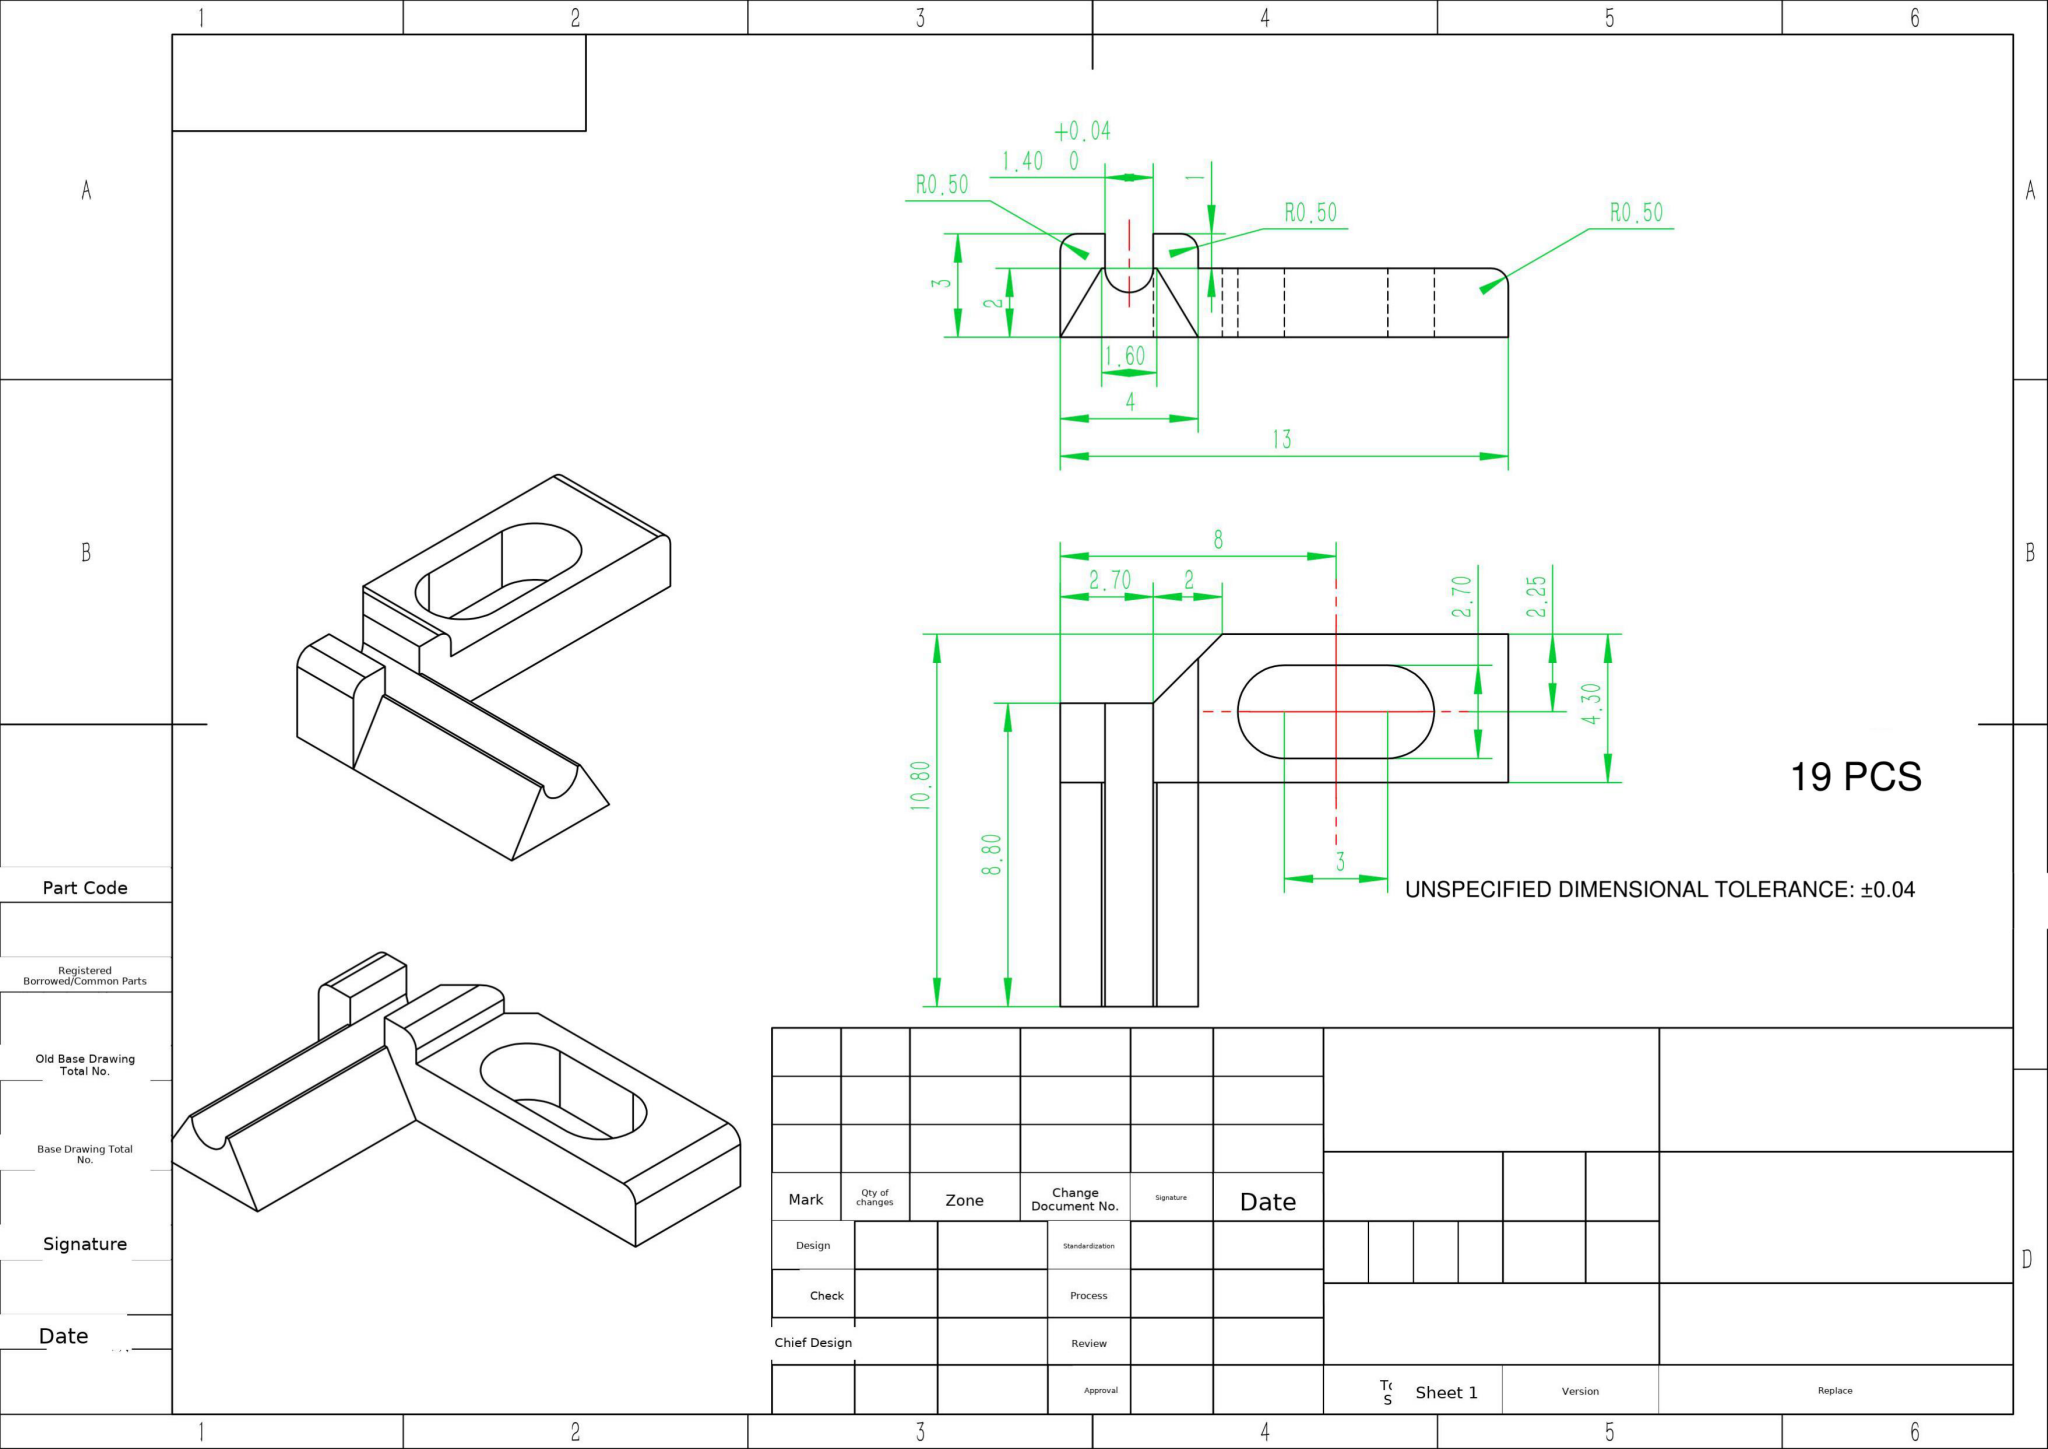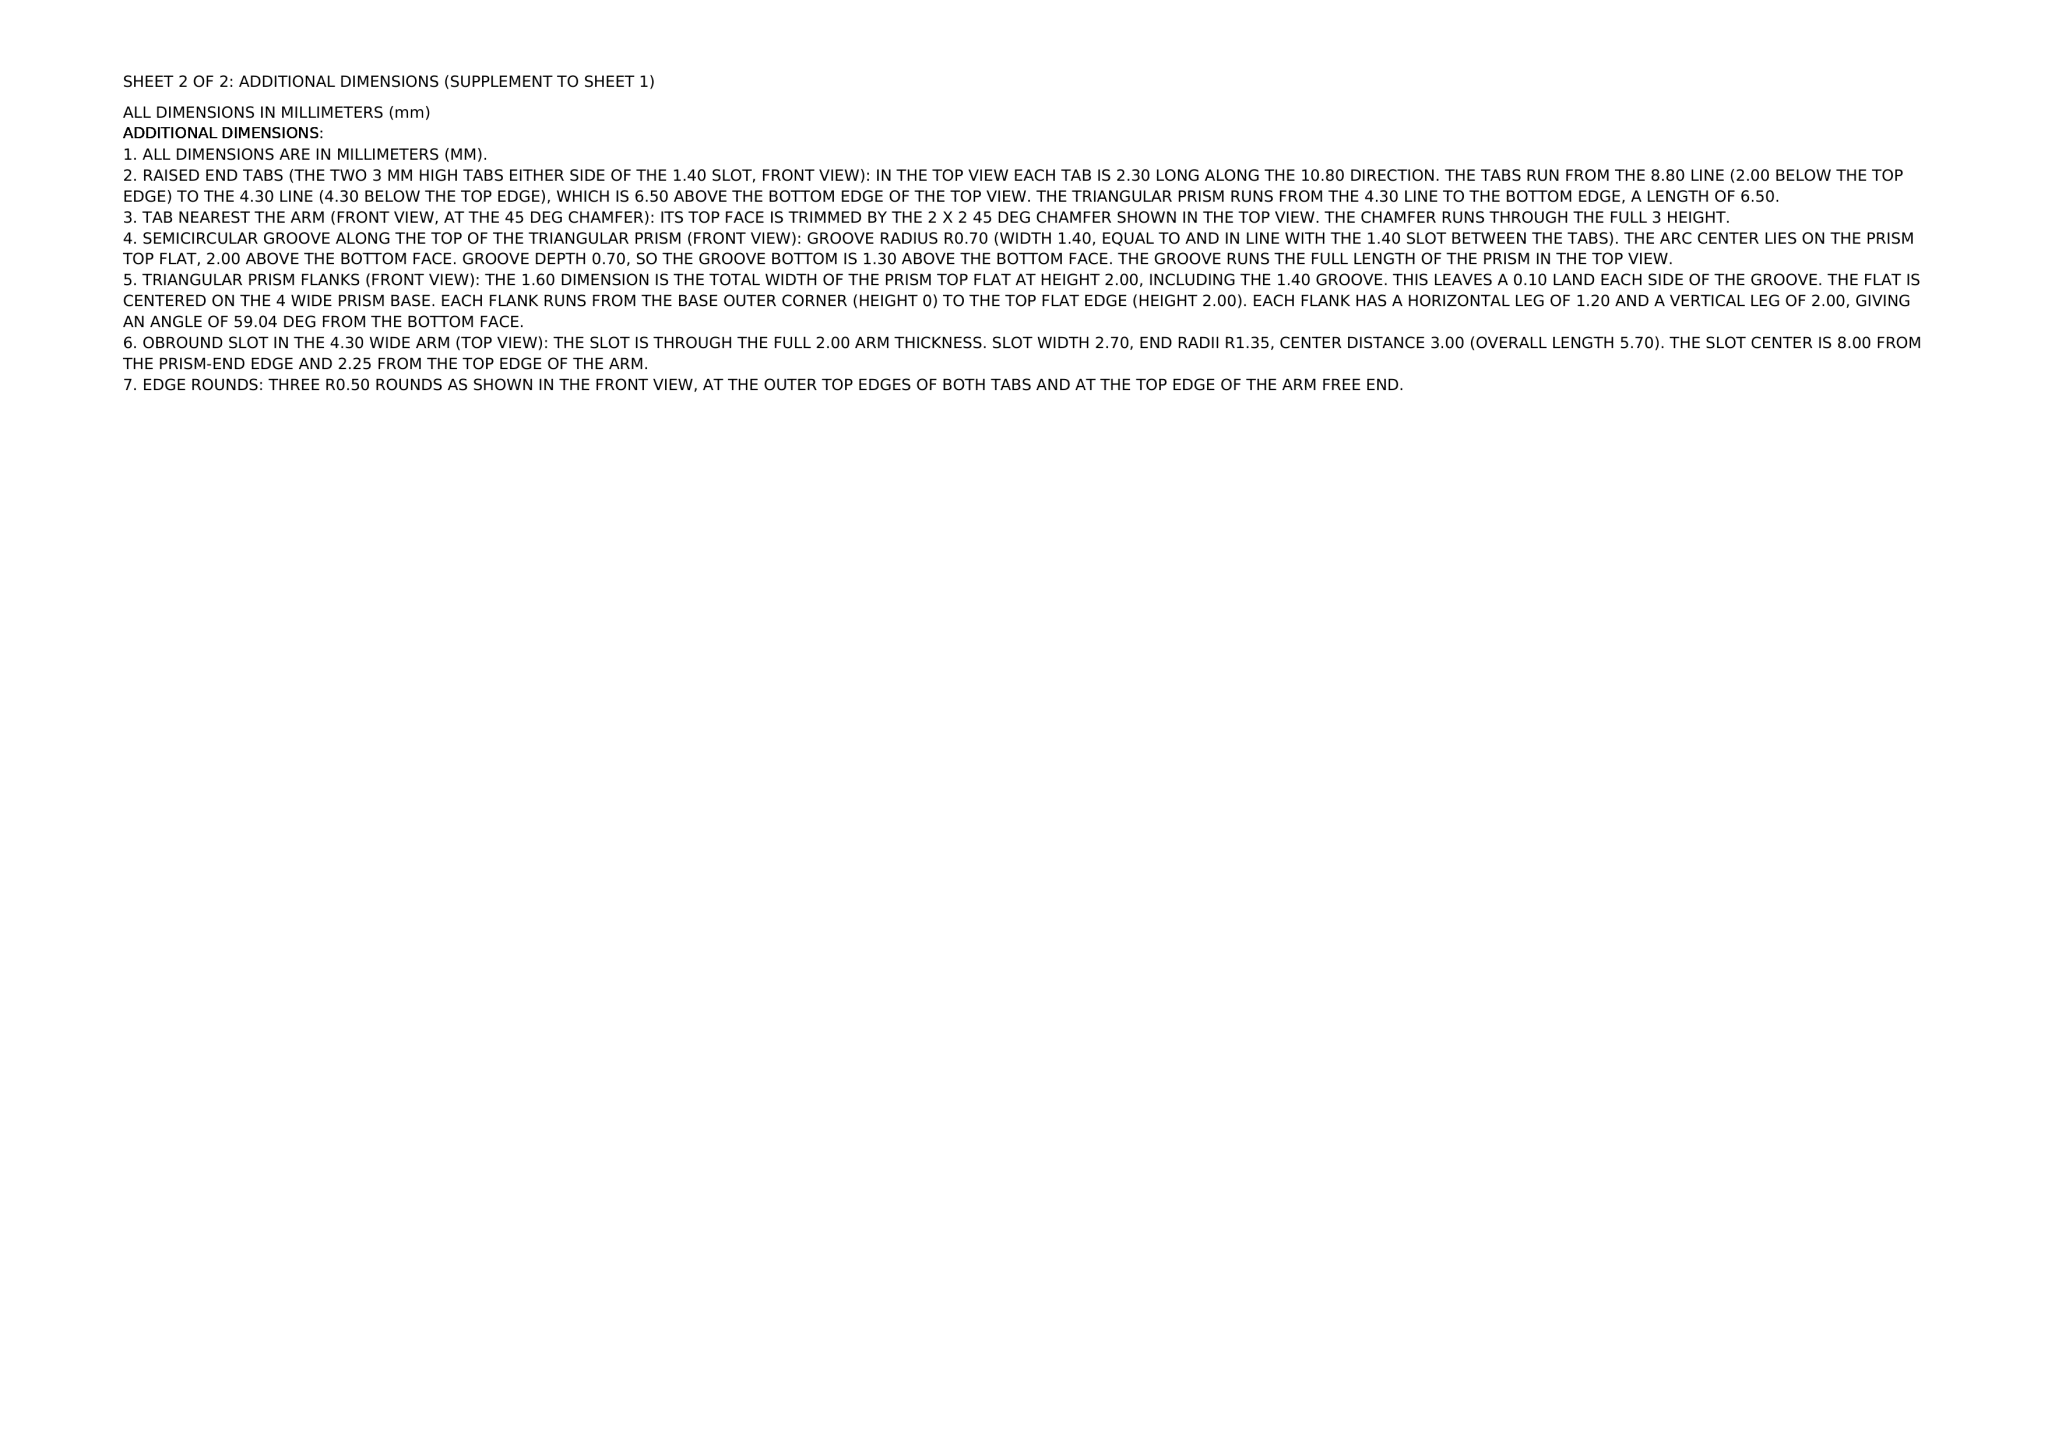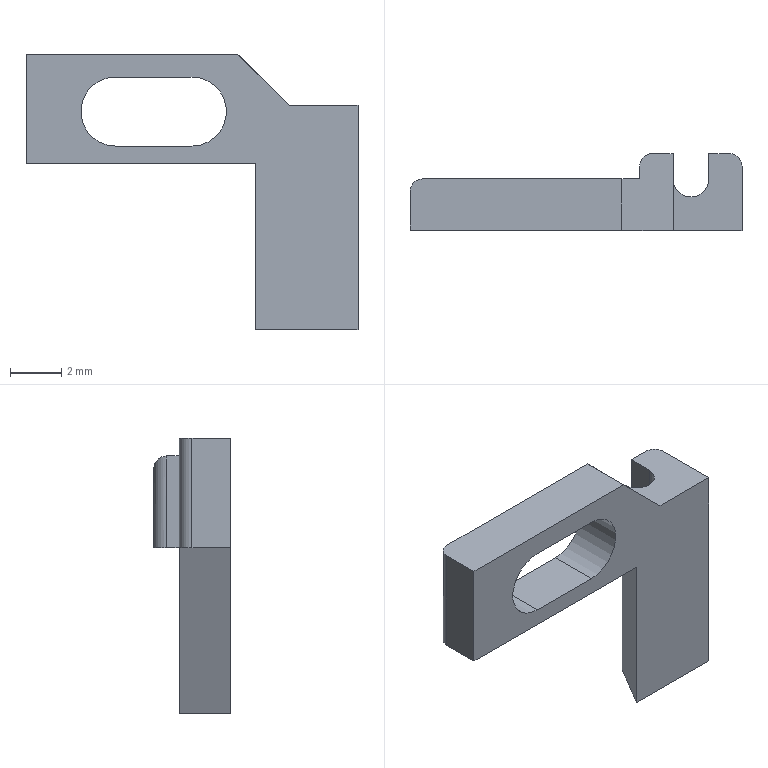Part | NX | mm | Offset Pedestal Clevis Bracket | 1 solid | 27 faces | box 13 x 3 x 10.8 mm | volume 105 mm3 | plane 21 | cylinder 6 | commonest cylinder face diameters 1 x3 2.7 x2 1.4 x1
STEP:
#1=COLOUR_RGB('',0.8431,0.,0.08627);
#2=FILL_AREA_STYLE_COLOUR('',#1);
#3=FILL_AREA_STYLE('',(#2));
#4=SURFACE_STYLE_FILL_AREA(#3);
#5=SURFACE_SIDE_STYLE('',(#4));
#6=SURFACE_STYLE_USAGE(.BOTH.,#5);
#7=PRESENTATION_STYLE_ASSIGNMENT((#6));
#8=CARTESIAN_POINT('',(9.,2.,-4.3));
#9=VERTEX_POINT('',#8);
#10=CARTESIAN_POINT('',(9.,2.5,-4.3));
#11=VERTEX_POINT('',#10);
#12=CARTESIAN_POINT('',(9.,2.,-4.3));
#13=DIRECTION('',(0.,1.,0.));
#14=VECTOR('',#13,1000.);
#15=LINE('',#12,#14);
#16=EDGE_CURVE('',#9,#11,#15,.T.);
#17=ORIENTED_EDGE('',*,*,#16,.T.);
#18=CARTESIAN_POINT('',(9.5,3.,-4.3));
#19=VERTEX_POINT('',#18);
#20=CARTESIAN_POINT('',(9.5,2.5,-4.3));
#21=DIRECTION('',(0.,0.,-1.));
#22=DIRECTION('',(1.,0.,0.));
#23=AXIS2_PLACEMENT_3D('',#20,#21,#22);
#24=CIRCLE('',#23,0.5);
#25=EDGE_CURVE('',#11,#19,#24,.T.);
#26=ORIENTED_EDGE('',*,*,#25,.T.);
#27=CARTESIAN_POINT('',(10.3,3.,-4.3));
#28=VERTEX_POINT('',#27);
#29=CARTESIAN_POINT('',(0.,3.,-4.3));
#30=DIRECTION('',(-1.,0.,0.));
#31=VECTOR('',#30,1000.);
#32=LINE('',#29,#31);
#33=EDGE_CURVE('',#28,#19,#32,.T.);
#34=ORIENTED_EDGE('',*,*,#33,.F.);
#35=CARTESIAN_POINT('',(10.3,2.,-4.3));
#36=VERTEX_POINT('',#35);
#37=CARTESIAN_POINT('',(10.3,2.,-4.3));
#38=DIRECTION('',(0.,-1.,0.));
#39=VECTOR('',#38,1000.);
#40=LINE('',#37,#39);
#41=EDGE_CURVE('',#28,#36,#40,.T.);
#42=ORIENTED_EDGE('',*,*,#41,.T.);
#43=CARTESIAN_POINT('',(10.2,2.,-4.3));
#44=VERTEX_POINT('',#43);
#45=CARTESIAN_POINT('',(0.,2.,-4.3));
#46=DIRECTION('',(-1.,0.,0.));
#47=VECTOR('',#46,1000.);
#48=LINE('',#45,#47);
#49=EDGE_CURVE('',#36,#44,#48,.T.);
#50=ORIENTED_EDGE('',*,*,#49,.T.);
#51=CARTESIAN_POINT('',(9.,0.,-4.3));
#52=VERTEX_POINT('',#51);
#53=CARTESIAN_POINT('',(7.5,-2.5,-4.3));
#54=DIRECTION('',(-0.5145,-0.8575,0.));
#55=VECTOR('',#54,1000.);
#56=LINE('',#53,#55);
#57=EDGE_CURVE('',#44,#52,#56,.T.);
#58=ORIENTED_EDGE('',*,*,#57,.T.);
#59=CARTESIAN_POINT('',(0.,0.,-4.3));
#60=VERTEX_POINT('',#59);
#61=CARTESIAN_POINT('',(0.,0.,-4.3));
#62=DIRECTION('',(-1.,0.,0.));
#63=VECTOR('',#62,1000.);
#64=LINE('',#61,#63);
#65=EDGE_CURVE('',#52,#60,#64,.T.);
#66=ORIENTED_EDGE('',*,*,#65,.T.);
#67=CARTESIAN_POINT('',(0.,1.5,-4.3));
#68=VERTEX_POINT('',#67);
#69=CARTESIAN_POINT('',(0.,2.,-4.3));
#70=DIRECTION('',(0.,-1.,0.));
#71=VECTOR('',#70,1000.);
#72=LINE('',#69,#71);
#73=EDGE_CURVE('',#68,#60,#72,.T.);
#74=ORIENTED_EDGE('',*,*,#73,.F.);
#75=CARTESIAN_POINT('',(0.5,2.,-4.3));
#76=VERTEX_POINT('',#75);
#77=CARTESIAN_POINT('',(0.5,1.5,-4.3));
#78=DIRECTION('',(0.,0.,-1.));
#79=DIRECTION('',(1.,0.,0.));
#80=AXIS2_PLACEMENT_3D('',#77,#78,#79);
#81=CIRCLE('',#80,0.5);
#82=EDGE_CURVE('',#68,#76,#81,.T.);
#83=ORIENTED_EDGE('',*,*,#82,.T.);
#84=CARTESIAN_POINT('',(0.,2.,-4.3));
#85=DIRECTION('',(-1.,0.,0.));
#86=VECTOR('',#85,1000.);
#87=LINE('',#84,#86);
#88=EDGE_CURVE('',#9,#76,#87,.T.);
#89=ORIENTED_EDGE('',*,*,#88,.F.);
#90=EDGE_LOOP('',(#17,#26,#34,#42,#50,#58,#66,#74,#83,#89));
#91=FACE_OUTER_BOUND('',#90,.T.);
#92=CARTESIAN_POINT('',(0.,2.,-4.3));
#93=DIRECTION('',(0.,0.,1.));
#94=DIRECTION('',(1.,0.,0.));
#95=AXIS2_PLACEMENT_3D('',#92,#93,#94);
#96=PLANE('',#95);
#97=ADVANCED_FACE('',(#91),#96,.F.);
#98=ORIENTED_EDGE('',*,*,#33,.T.);
#99=CARTESIAN_POINT('',(9.5,3.,-1.2));
#100=VERTEX_POINT('',#99);
#101=CARTESIAN_POINT('',(9.5,3.,-0.7));
#102=DIRECTION('',(0.,0.,1.));
#103=VECTOR('',#102,1000.);
#104=LINE('',#101,#103);
#105=EDGE_CURVE('',#19,#100,#104,.T.);
#106=ORIENTED_EDGE('',*,*,#105,.T.);
#107=CARTESIAN_POINT('',(10.3,3.,-2.));
#108=VERTEX_POINT('',#107);
#109=CARTESIAN_POINT('',(8.3,3.,0.));
#110=DIRECTION('',(0.7071,0.,-0.7071));
#111=VECTOR('',#110,1000.);
#112=LINE('',#109,#111);
#113=EDGE_CURVE('',#100,#108,#112,.T.);
#114=ORIENTED_EDGE('',*,*,#113,.T.);
#115=CARTESIAN_POINT('',(10.3,3.,-8.));
#116=DIRECTION('',(0.,0.,1.));
#117=VECTOR('',#116,1000.);
#118=LINE('',#115,#117);
#119=EDGE_CURVE('',#28,#108,#118,.T.);
#120=ORIENTED_EDGE('',*,*,#119,.F.);
#121=EDGE_LOOP('',(#98,#106,#114,#120));
#122=FACE_OUTER_BOUND('',#121,.T.);
#123=CARTESIAN_POINT('',(0.,3.,0.));
#124=DIRECTION('',(0.,1.,0.));
#125=DIRECTION('',(0.,0.,1.));
#126=AXIS2_PLACEMENT_3D('',#123,#124,#125);
#127=PLANE('',#126);
#128=ADVANCED_FACE('',(#122),#127,.T.);
#129=CARTESIAN_POINT('',(11.8,2.,-4.3));
#130=VERTEX_POINT('',#129);
#131=CARTESIAN_POINT('',(11.7,2.,-4.3));
#132=VERTEX_POINT('',#131);
#133=CARTESIAN_POINT('',(0.,2.,-4.3));
#134=DIRECTION('',(-1.,0.,0.));
#135=VECTOR('',#134,1000.);
#136=LINE('',#133,#135);
#137=EDGE_CURVE('',#130,#132,#136,.T.);
#138=ORIENTED_EDGE('',*,*,#137,.F.);
#139=CARTESIAN_POINT('',(11.8,2.,-10.8));
#140=VERTEX_POINT('',#139);
#141=CARTESIAN_POINT('',(11.8,2.,-0.));
#142=DIRECTION('',(-0.,0.,-1.));
#143=VECTOR('',#142,1000.);
#144=LINE('',#141,#143);
#145=EDGE_CURVE('',#130,#140,#144,.T.);
#146=ORIENTED_EDGE('',*,*,#145,.T.);
#147=CARTESIAN_POINT('',(11.7,2.,-10.8));
#148=VERTEX_POINT('',#147);
#149=CARTESIAN_POINT('',(11.7,2.,-10.8));
#150=DIRECTION('',(1.,0.,0.));
#151=VECTOR('',#150,1000.);
#152=LINE('',#149,#151);
#153=EDGE_CURVE('',#148,#140,#152,.T.);
#154=ORIENTED_EDGE('',*,*,#153,.F.);
#155=CARTESIAN_POINT('',(11.7,2.,5.7));
#156=DIRECTION('',(0.,0.,-1.));
#157=VECTOR('',#156,1000.);
#158=LINE('',#155,#157);
#159=EDGE_CURVE('',#132,#148,#158,.T.);
#160=ORIENTED_EDGE('',*,*,#159,.F.);
#161=EDGE_LOOP('',(#138,#146,#154,#160));
#162=FACE_OUTER_BOUND('',#161,.T.);
#163=CARTESIAN_POINT('',(0.,2.,0.));
#164=DIRECTION('',(0.,-1.,0.));
#165=DIRECTION('',(0.,0.,-1.));
#166=AXIS2_PLACEMENT_3D('',#163,#164,#165);
#167=PLANE('',#166);
#168=ADVANCED_FACE('',(#162),#167,.F.);
#169=CARTESIAN_POINT('',(10.2,2.,-10.8));
#170=VERTEX_POINT('',#169);
#171=CARTESIAN_POINT('',(10.3,2.,-10.8));
#172=VERTEX_POINT('',#171);
#173=CARTESIAN_POINT('',(9.,2.,-10.8));
#174=DIRECTION('',(1.,-0.,0.));
#175=VECTOR('',#174,1000.);
#176=LINE('',#173,#175);
#177=EDGE_CURVE('',#170,#172,#176,.T.);
#178=ORIENTED_EDGE('',*,*,#177,.F.);
#179=CARTESIAN_POINT('',(10.2,2.,0.));
#180=DIRECTION('',(0.,0.,1.));
#181=VECTOR('',#180,1000.);
#182=LINE('',#179,#181);
#183=EDGE_CURVE('',#170,#44,#182,.T.);
#184=ORIENTED_EDGE('',*,*,#183,.T.);
#185=ORIENTED_EDGE('',*,*,#49,.F.);
#186=CARTESIAN_POINT('',(10.3,2.,5.7));
#187=DIRECTION('',(0.,0.,-1.));
#188=VECTOR('',#187,1000.);
#189=LINE('',#186,#188);
#190=EDGE_CURVE('',#36,#172,#189,.T.);
#191=ORIENTED_EDGE('',*,*,#190,.T.);
#192=EDGE_LOOP('',(#178,#184,#185,#191));
#193=FACE_OUTER_BOUND('',#192,.T.);
#194=CARTESIAN_POINT('',(0.,2.,0.));
#195=DIRECTION('',(0.,-1.,0.));
#196=DIRECTION('',(0.,0.,-1.));
#197=AXIS2_PLACEMENT_3D('',#194,#195,#196);
#198=PLANE('',#197);
#199=ADVANCED_FACE('',(#193),#198,.F.);
#200=CARTESIAN_POINT('',(12.5,3.,-4.3));
#201=VERTEX_POINT('',#200);
#202=CARTESIAN_POINT('',(11.7,3.,-4.3));
#203=VERTEX_POINT('',#202);
#204=CARTESIAN_POINT('',(0.,3.,-4.3));
#205=DIRECTION('',(-1.,0.,0.));
#206=VECTOR('',#205,1000.);
#207=LINE('',#204,#206);
#208=EDGE_CURVE('',#201,#203,#207,.T.);
#209=ORIENTED_EDGE('',*,*,#208,.F.);
#210=CARTESIAN_POINT('',(13.,2.5,-4.3));
#211=VERTEX_POINT('',#210);
#212=CARTESIAN_POINT('',(12.5,2.5,-4.3));
#213=DIRECTION('',(0.,0.,-1.));
#214=DIRECTION('',(1.,0.,0.));
#215=AXIS2_PLACEMENT_3D('',#212,#213,#214);
#216=CIRCLE('',#215,0.5);
#217=EDGE_CURVE('',#201,#211,#216,.T.);
#218=ORIENTED_EDGE('',*,*,#217,.T.);
#219=CARTESIAN_POINT('',(13.,0.,-4.3));
#220=VERTEX_POINT('',#219);
#221=CARTESIAN_POINT('',(13.,3.,-4.3));
#222=DIRECTION('',(0.,-1.,0.));
#223=VECTOR('',#222,1000.);
#224=LINE('',#221,#223);
#225=EDGE_CURVE('',#211,#220,#224,.T.);
#226=ORIENTED_EDGE('',*,*,#225,.T.);
#227=CARTESIAN_POINT('',(8.676,7.206,-4.3));
#228=DIRECTION('',(-0.5145,0.8575,0.));
#229=VECTOR('',#228,1000.);
#230=LINE('',#227,#229);
#231=EDGE_CURVE('',#220,#130,#230,.T.);
#232=ORIENTED_EDGE('',*,*,#231,.T.);
#233=ORIENTED_EDGE('',*,*,#137,.T.);
#234=CARTESIAN_POINT('',(11.7,2.,-4.3));
#235=DIRECTION('',(0.,1.,0.));
#236=VECTOR('',#235,1000.);
#237=LINE('',#234,#236);
#238=EDGE_CURVE('',#132,#203,#237,.T.);
#239=ORIENTED_EDGE('',*,*,#238,.T.);
#240=EDGE_LOOP('',(#209,#218,#226,#232,#233,#239));
#241=FACE_OUTER_BOUND('',#240,.T.);
#242=CARTESIAN_POINT('',(0.,2.,-4.3));
#243=DIRECTION('',(0.,0.,1.));
#244=DIRECTION('',(1.,0.,0.));
#245=AXIS2_PLACEMENT_3D('',#242,#243,#244);
#246=PLANE('',#245);
#247=ADVANCED_FACE('',(#241),#246,.F.);
#248=CARTESIAN_POINT('',(0.,1.5,0.));
#249=VERTEX_POINT('',#248);
#250=CARTESIAN_POINT('',(0.,0.,0.));
#251=VERTEX_POINT('',#250);
#252=CARTESIAN_POINT('',(0.,2.,0.));
#253=DIRECTION('',(0.,-1.,0.));
#254=VECTOR('',#253,1000.);
#255=LINE('',#252,#254);
#256=EDGE_CURVE('',#249,#251,#255,.T.);
#257=ORIENTED_EDGE('',*,*,#256,.F.);
#258=CARTESIAN_POINT('',(0.,1.5,0.));
#259=DIRECTION('',(0.,0.,-1.));
#260=VECTOR('',#259,1000.);
#261=LINE('',#258,#260);
#262=EDGE_CURVE('',#249,#68,#261,.T.);
#263=ORIENTED_EDGE('',*,*,#262,.T.);
#264=ORIENTED_EDGE('',*,*,#73,.T.);
#265=CARTESIAN_POINT('',(0.,0.,0.));
#266=DIRECTION('',(0.,0.,1.));
#267=VECTOR('',#266,1000.);
#268=LINE('',#265,#267);
#269=EDGE_CURVE('',#60,#251,#268,.T.);
#270=ORIENTED_EDGE('',*,*,#269,.T.);
#271=EDGE_LOOP('',(#257,#263,#264,#270));
#272=FACE_OUTER_BOUND('',#271,.T.);
#273=CARTESIAN_POINT('',(0.,2.,0.));
#274=DIRECTION('',(1.,0.,0.));
#275=DIRECTION('',(0.,0.,-1.));
#276=AXIS2_PLACEMENT_3D('',#273,#274,#275);
#277=PLANE('',#276);
#278=ADVANCED_FACE('',(#272),#277,.F.);
#279=CARTESIAN_POINT('',(0.5,2.,0.));
#280=VERTEX_POINT('',#279);
#281=CARTESIAN_POINT('',(8.3,2.,0.));
#282=VERTEX_POINT('',#281);
#283=CARTESIAN_POINT('',(0.,2.,0.));
#284=DIRECTION('',(1.,0.,0.));
#285=VECTOR('',#284,1000.);
#286=LINE('',#283,#285);
#287=EDGE_CURVE('',#280,#282,#286,.T.);
#288=ORIENTED_EDGE('',*,*,#287,.F.);
#289=CARTESIAN_POINT('',(0.5,1.5,0.));
#290=DIRECTION('',(0.,0.,1.));
#291=DIRECTION('',(-1.,0.,0.));
#292=AXIS2_PLACEMENT_3D('',#289,#290,#291);
#293=CIRCLE('',#292,0.5);
#294=EDGE_CURVE('',#280,#249,#293,.T.);
#295=ORIENTED_EDGE('',*,*,#294,.T.);
#296=ORIENTED_EDGE('',*,*,#256,.T.);
#297=CARTESIAN_POINT('',(8.3,0.,0.));
#298=VERTEX_POINT('',#297);
#299=CARTESIAN_POINT('',(0.,0.,0.));
#300=DIRECTION('',(1.,0.,0.));
#301=VECTOR('',#300,1000.);
#302=LINE('',#299,#301);
#303=EDGE_CURVE('',#251,#298,#302,.T.);
#304=ORIENTED_EDGE('',*,*,#303,.T.);
#305=CARTESIAN_POINT('',(8.3,2.,0.));
#306=DIRECTION('',(0.,1.,0.));
#307=VECTOR('',#306,1000.);
#308=LINE('',#305,#307);
#309=EDGE_CURVE('',#298,#282,#308,.T.);
#310=ORIENTED_EDGE('',*,*,#309,.T.);
#311=EDGE_LOOP('',(#288,#295,#296,#304,#310));
#312=FACE_OUTER_BOUND('',#311,.T.);
#313=CARTESIAN_POINT('',(0.,2.,0.));
#314=DIRECTION('',(0.,0.,-1.));
#315=DIRECTION('',(-1.,0.,0.));
#316=AXIS2_PLACEMENT_3D('',#313,#314,#315);
#317=PLANE('',#316);
#318=ADVANCED_FACE('',(#312),#317,.F.);
#319=CARTESIAN_POINT('',(13.,0.,-2.));
#320=VERTEX_POINT('',#319);
#321=CARTESIAN_POINT('',(13.,0.,-0.));
#322=DIRECTION('',(-0.,0.,-1.));
#323=VECTOR('',#322,1000.);
#324=LINE('',#321,#323);
#325=EDGE_CURVE('',#320,#220,#324,.T.);
#326=ORIENTED_EDGE('',*,*,#325,.F.);
#327=CARTESIAN_POINT('',(10.3,0.,-2.));
#328=VERTEX_POINT('',#327);
#329=CARTESIAN_POINT('',(-0.,0.,-2.));
#330=DIRECTION('',(1.,0.,-0.));
#331=VECTOR('',#330,1000.);
#332=LINE('',#329,#331);
#333=EDGE_CURVE('',#328,#320,#332,.T.);
#334=ORIENTED_EDGE('',*,*,#333,.F.);
#335=CARTESIAN_POINT('',(4.15,0.,4.15));
#336=DIRECTION('',(-0.7071,0.,0.7071));
#337=VECTOR('',#336,1000.);
#338=LINE('',#335,#337);
#339=EDGE_CURVE('',#328,#298,#338,.T.);
#340=ORIENTED_EDGE('',*,*,#339,.T.);
#341=ORIENTED_EDGE('',*,*,#303,.F.);
#342=ORIENTED_EDGE('',*,*,#269,.F.);
#343=ORIENTED_EDGE('',*,*,#65,.F.);
#344=CARTESIAN_POINT('',(9.,0.,-10.8));
#345=VERTEX_POINT('',#344);
#346=CARTESIAN_POINT('',(9.,0.,-10.8));
#347=DIRECTION('',(0.,0.,1.));
#348=VECTOR('',#347,1000.);
#349=LINE('',#346,#348);
#350=EDGE_CURVE('',#345,#52,#349,.T.);
#351=ORIENTED_EDGE('',*,*,#350,.F.);
#352=CARTESIAN_POINT('',(13.,-0.,-10.8));
#353=VERTEX_POINT('',#352);
#354=CARTESIAN_POINT('',(13.,-0.,-10.8));
#355=DIRECTION('',(-1.,0.,0.));
#356=VECTOR('',#355,1000.);
#357=LINE('',#354,#356);
#358=EDGE_CURVE('',#353,#345,#357,.T.);
#359=ORIENTED_EDGE('',*,*,#358,.F.);
#360=CARTESIAN_POINT('',(13.,0.,-0.));
#361=DIRECTION('',(-0.,0.,-1.));
#362=VECTOR('',#361,1000.);
#363=LINE('',#360,#362);
#364=EDGE_CURVE('',#220,#353,#363,.T.);
#365=ORIENTED_EDGE('',*,*,#364,.F.);
#366=EDGE_LOOP('',(#326,#334,#340,#341,#342,#343,#351,#359,#365));
#367=FACE_OUTER_BOUND('',#366,.T.);
#368=CARTESIAN_POINT('',(6.5,0.,-3.6));
#369=VERTEX_POINT('',#368);
#370=CARTESIAN_POINT('',(6.5,0.,-0.9));
#371=VERTEX_POINT('',#370);
#372=CARTESIAN_POINT('',(6.5,0.,-2.25));
#373=DIRECTION('',(0.,-1.,0.));
#374=DIRECTION('',(0.,0.,-1.));
#375=AXIS2_PLACEMENT_3D('',#372,#373,#374);
#376=CIRCLE('',#375,1.35);
#377=EDGE_CURVE('',#369,#371,#376,.T.);
#378=ORIENTED_EDGE('',*,*,#377,.F.);
#379=CARTESIAN_POINT('',(3.5,0.,-3.6));
#380=VERTEX_POINT('',#379);
#381=CARTESIAN_POINT('',(-0.,0.,-3.6));
#382=DIRECTION('',(1.,0.,-0.));
#383=VECTOR('',#382,1000.);
#384=LINE('',#381,#383);
#385=EDGE_CURVE('',#380,#369,#384,.T.);
#386=ORIENTED_EDGE('',*,*,#385,.F.);
#387=CARTESIAN_POINT('',(3.5,0.,-0.9));
#388=VERTEX_POINT('',#387);
#389=CARTESIAN_POINT('',(3.5,0.,-2.25));
#390=DIRECTION('',(0.,-1.,0.));
#391=DIRECTION('',(0.,0.,-1.));
#392=AXIS2_PLACEMENT_3D('',#389,#390,#391);
#393=CIRCLE('',#392,1.35);
#394=EDGE_CURVE('',#388,#380,#393,.T.);
#395=ORIENTED_EDGE('',*,*,#394,.F.);
#396=CARTESIAN_POINT('',(-0.,0.,-0.9));
#397=DIRECTION('',(-1.,0.,0.));
#398=VECTOR('',#397,1000.);
#399=LINE('',#396,#398);
#400=EDGE_CURVE('',#371,#388,#399,.T.);
#401=ORIENTED_EDGE('',*,*,#400,.F.);
#402=EDGE_LOOP('',(#378,#386,#395,#401));
#403=FACE_BOUND('',#402,.T.);
#404=CARTESIAN_POINT('',(0.,0.,0.));
#405=DIRECTION('',(0.,-1.,0.));
#406=DIRECTION('',(0.,0.,-1.));
#407=AXIS2_PLACEMENT_3D('',#404,#405,#406);
#408=PLANE('',#407);
#409=ADVANCED_FACE('',(#367,#403),#408,.T.);
#410=CARTESIAN_POINT('',(13.,2.5,-2.));
#411=VERTEX_POINT('',#410);
#412=CARTESIAN_POINT('',(13.,-8.,-2.));
#413=DIRECTION('',(0.,1.,0.));
#414=VECTOR('',#413,1000.);
#415=LINE('',#412,#414);
#416=EDGE_CURVE('',#320,#411,#415,.T.);
#417=ORIENTED_EDGE('',*,*,#416,.T.);
#418=CARTESIAN_POINT('',(12.5,3.,-2.));
#419=VERTEX_POINT('',#418);
#420=CARTESIAN_POINT('',(12.5,2.5,-2.));
#421=DIRECTION('',(0.,0.,1.));
#422=DIRECTION('',(-1.,0.,0.));
#423=AXIS2_PLACEMENT_3D('',#420,#421,#422);
#424=CIRCLE('',#423,0.5);
#425=EDGE_CURVE('',#411,#419,#424,.T.);
#426=ORIENTED_EDGE('',*,*,#425,.T.);
#427=CARTESIAN_POINT('',(11.7,3.,-2.));
#428=VERTEX_POINT('',#427);
#429=CARTESIAN_POINT('',(13.,3.,-2.));
#430=DIRECTION('',(1.,0.,-0.));
#431=VECTOR('',#430,1000.);
#432=LINE('',#429,#431);
#433=EDGE_CURVE('',#428,#419,#432,.T.);
#434=ORIENTED_EDGE('',*,*,#433,.F.);
#435=CARTESIAN_POINT('',(11.7,2.,-2.));
#436=VERTEX_POINT('',#435);
#437=CARTESIAN_POINT('',(11.7,3.,-2.));
#438=DIRECTION('',(0.,1.,0.));
#439=VECTOR('',#438,1000.);
#440=LINE('',#437,#439);
#441=EDGE_CURVE('',#436,#428,#440,.T.);
#442=ORIENTED_EDGE('',*,*,#441,.F.);
#443=CARTESIAN_POINT('',(10.3,2.,-2.));
#444=VERTEX_POINT('',#443);
#445=CARTESIAN_POINT('',(11.,2.,-2.));
#446=DIRECTION('',(-0.,0.,-1.));
#447=DIRECTION('',(-1.,0.,0.));
#448=AXIS2_PLACEMENT_3D('',#445,#446,#447);
#449=CIRCLE('',#448,0.7);
#450=EDGE_CURVE('',#436,#444,#449,.T.);
#451=ORIENTED_EDGE('',*,*,#450,.T.);
#452=CARTESIAN_POINT('',(10.3,-8.,-2.));
#453=DIRECTION('',(0.,1.,0.));
#454=VECTOR('',#453,1000.);
#455=LINE('',#452,#454);
#456=EDGE_CURVE('',#328,#444,#455,.T.);
#457=ORIENTED_EDGE('',*,*,#456,.F.);
#458=ORIENTED_EDGE('',*,*,#333,.T.);
#459=EDGE_LOOP('',(#417,#426,#434,#442,#451,#457,#458));
#460=FACE_OUTER_BOUND('',#459,.T.);
#461=CARTESIAN_POINT('',(17.5,-8.,-2.));
#462=DIRECTION('',(-0.,0.,-1.));
#463=DIRECTION('',(-1.,0.,0.));
#464=AXIS2_PLACEMENT_3D('',#461,#462,#463);
#465=PLANE('',#464);
#466=ADVANCED_FACE('',(#460),#465,.F.);
#467=ORIENTED_EDGE('',*,*,#159,.T.);
#468=CARTESIAN_POINT('',(11.,2.,-10.8));
#469=DIRECTION('',(0.,0.,1.));
#470=DIRECTION('',(-1.,0.,0.));
#471=AXIS2_PLACEMENT_3D('',#468,#469,#470);
#472=CIRCLE('',#471,0.7);
#473=EDGE_CURVE('',#172,#148,#472,.T.);
#474=ORIENTED_EDGE('',*,*,#473,.F.);
#475=ORIENTED_EDGE('',*,*,#190,.F.);
#476=CARTESIAN_POINT('',(10.3,2.,5.7));
#477=DIRECTION('',(0.,0.,-1.));
#478=VECTOR('',#477,1000.);
#479=LINE('',#476,#478);
#480=EDGE_CURVE('',#444,#36,#479,.T.);
#481=ORIENTED_EDGE('',*,*,#480,.F.);
#482=ORIENTED_EDGE('',*,*,#450,.F.);
#483=CARTESIAN_POINT('',(11.7,2.,5.7));
#484=DIRECTION('',(0.,0.,-1.));
#485=VECTOR('',#484,1000.);
#486=LINE('',#483,#485);
#487=EDGE_CURVE('',#436,#132,#486,.T.);
#488=ORIENTED_EDGE('',*,*,#487,.T.);
#489=EDGE_LOOP('',(#467,#474,#475,#481,#482,#488));
#490=FACE_OUTER_BOUND('',#489,.T.);
#491=CARTESIAN_POINT('',(11.,2.,5.7));
#492=DIRECTION('',(0.,0.,-1.));
#493=DIRECTION('',(-1.,0.,0.));
#494=AXIS2_PLACEMENT_3D('',#491,#492,#493);
#495=CYLINDRICAL_SURFACE('',#494,0.7);
#496=ADVANCED_FACE('',(#490),#495,.F.);
#497=ORIENTED_EDGE('',*,*,#377,.T.);
#498=CARTESIAN_POINT('',(6.5,2.,-0.9));
#499=VERTEX_POINT('',#498);
#500=CARTESIAN_POINT('',(6.5,-3.,-0.9));
#501=DIRECTION('',(0.,1.,0.));
#502=VECTOR('',#501,1000.);
#503=LINE('',#500,#502);
#504=EDGE_CURVE('',#371,#499,#503,.T.);
#505=ORIENTED_EDGE('',*,*,#504,.T.);
#506=CARTESIAN_POINT('',(6.5,2.,-3.6));
#507=VERTEX_POINT('',#506);
#508=CARTESIAN_POINT('',(6.5,2.,-2.25));
#509=DIRECTION('',(0.,1.,0.));
#510=DIRECTION('',(0.,0.,1.));
#511=AXIS2_PLACEMENT_3D('',#508,#509,#510);
#512=CIRCLE('',#511,1.35);
#513=EDGE_CURVE('',#499,#507,#512,.T.);
#514=ORIENTED_EDGE('',*,*,#513,.T.);
#515=CARTESIAN_POINT('',(6.5,-3.,-3.6));
#516=DIRECTION('',(0.,1.,0.));
#517=VECTOR('',#516,1000.);
#518=LINE('',#515,#517);
#519=EDGE_CURVE('',#369,#507,#518,.T.);
#520=ORIENTED_EDGE('',*,*,#519,.F.);
#521=EDGE_LOOP('',(#497,#505,#514,#520));
#522=FACE_OUTER_BOUND('',#521,.T.);
#523=CARTESIAN_POINT('',(6.5,-3.,-2.25));
#524=DIRECTION('',(0.,1.,0.));
#525=DIRECTION('',(0.,0.,1.));
#526=AXIS2_PLACEMENT_3D('',#523,#524,#525);
#527=CYLINDRICAL_SURFACE('',#526,1.35);
#528=ADVANCED_FACE('',(#522),#527,.F.);
#529=ORIENTED_EDGE('',*,*,#400,.T.);
#530=CARTESIAN_POINT('',(3.5,2.,-0.9));
#531=VERTEX_POINT('',#530);
#532=CARTESIAN_POINT('',(3.5,-3.,-0.9));
#533=DIRECTION('',(0.,1.,0.));
#534=VECTOR('',#533,1000.);
#535=LINE('',#532,#534);
#536=EDGE_CURVE('',#388,#531,#535,.T.);
#537=ORIENTED_EDGE('',*,*,#536,.T.);
#538=CARTESIAN_POINT('',(6.5,2.,-0.9));
#539=DIRECTION('',(1.,0.,-0.));
#540=VECTOR('',#539,1000.);
#541=LINE('',#538,#540);
#542=EDGE_CURVE('',#531,#499,#541,.T.);
#543=ORIENTED_EDGE('',*,*,#542,.T.);
#544=ORIENTED_EDGE('',*,*,#504,.F.);
#545=EDGE_LOOP('',(#529,#537,#543,#544));
#546=FACE_OUTER_BOUND('',#545,.T.);
#547=CARTESIAN_POINT('',(6.5,-3.,-0.9));
#548=DIRECTION('',(0.,0.,1.));
#549=DIRECTION('',(1.,0.,-0.));
#550=AXIS2_PLACEMENT_3D('',#547,#548,#549);
#551=PLANE('',#550);
#552=ADVANCED_FACE('',(#546),#551,.F.);
#553=ORIENTED_EDGE('',*,*,#394,.T.);
#554=CARTESIAN_POINT('',(3.5,2.,-3.6));
#555=VERTEX_POINT('',#554);
#556=CARTESIAN_POINT('',(3.5,-3.,-3.6));
#557=DIRECTION('',(0.,1.,0.));
#558=VECTOR('',#557,1000.);
#559=LINE('',#556,#558);
#560=EDGE_CURVE('',#380,#555,#559,.T.);
#561=ORIENTED_EDGE('',*,*,#560,.T.);
#562=CARTESIAN_POINT('',(3.5,2.,-2.25));
#563=DIRECTION('',(0.,1.,0.));
#564=DIRECTION('',(0.,0.,1.));
#565=AXIS2_PLACEMENT_3D('',#562,#563,#564);
#566=CIRCLE('',#565,1.35);
#567=EDGE_CURVE('',#555,#531,#566,.T.);
#568=ORIENTED_EDGE('',*,*,#567,.T.);
#569=ORIENTED_EDGE('',*,*,#536,.F.);
#570=EDGE_LOOP('',(#553,#561,#568,#569));
#571=FACE_OUTER_BOUND('',#570,.T.);
#572=CARTESIAN_POINT('',(3.5,-3.,-2.25));
#573=DIRECTION('',(0.,1.,0.));
#574=DIRECTION('',(0.,0.,1.));
#575=AXIS2_PLACEMENT_3D('',#572,#573,#574);
#576=CYLINDRICAL_SURFACE('',#575,1.35);
#577=ADVANCED_FACE('',(#571),#576,.F.);
#578=ORIENTED_EDGE('',*,*,#385,.T.);
#579=ORIENTED_EDGE('',*,*,#519,.T.);
#580=CARTESIAN_POINT('',(6.5,2.,-3.6));
#581=DIRECTION('',(-1.,0.,0.));
#582=VECTOR('',#581,1000.);
#583=LINE('',#580,#582);
#584=EDGE_CURVE('',#507,#555,#583,.T.);
#585=ORIENTED_EDGE('',*,*,#584,.T.);
#586=ORIENTED_EDGE('',*,*,#560,.F.);
#587=EDGE_LOOP('',(#578,#579,#585,#586));
#588=FACE_OUTER_BOUND('',#587,.T.);
#589=CARTESIAN_POINT('',(6.5,-3.,-3.6));
#590=DIRECTION('',(-0.,0.,-1.));
#591=DIRECTION('',(-1.,0.,0.));
#592=AXIS2_PLACEMENT_3D('',#589,#590,#591);
#593=PLANE('',#592);
#594=ADVANCED_FACE('',(#588),#593,.F.);
#595=ORIENTED_EDGE('',*,*,#113,.F.);
#596=CARTESIAN_POINT('',(9.,2.5,-0.7));
#597=VERTEX_POINT('',#596);
#598=CARTESIAN_POINT('',(9.5,3.,-1.2));
#599=CARTESIAN_POINT('',(9.207,3.,-0.9071));
#600=CARTESIAN_POINT('',(9.,2.793,-0.7));
#601=CARTESIAN_POINT('',(9.,2.5,-0.7));
#602=(BOUNDED_CURVE()B_SPLINE_CURVE(3,(#598,#599,#600,#601),.UNSPECIFIED.,.F.,.T.)B_SPLINE_CURVE_WITH_KNOTS((4,4),(4.712,6.283),.UNSPECIFIED.)CURVE()GEOMETRIC_REPRESENTATION_ITEM()RATIONAL_B_SPLINE_CURVE((1.,0.8047,0.8047,1.))REPRESENTATION_ITEM(''));
#603=EDGE_CURVE('',#100,#597,#602,.T.);
#604=ORIENTED_EDGE('',*,*,#603,.T.);
#605=CARTESIAN_POINT('',(9.,2.,-0.7));
#606=VERTEX_POINT('',#605);
#607=CARTESIAN_POINT('',(9.,2.,-0.7));
#608=DIRECTION('',(0.,1.,0.));
#609=VECTOR('',#608,1000.);
#610=LINE('',#607,#609);
#611=EDGE_CURVE('',#606,#597,#610,.T.);
#612=ORIENTED_EDGE('',*,*,#611,.F.);
#613=CARTESIAN_POINT('',(8.3,2.,0.));
#614=DIRECTION('',(0.7071,0.,-0.7071));
#615=VECTOR('',#614,1000.);
#616=LINE('',#613,#615);
#617=EDGE_CURVE('',#282,#606,#616,.T.);
#618=ORIENTED_EDGE('',*,*,#617,.F.);
#619=ORIENTED_EDGE('',*,*,#309,.F.);
#620=ORIENTED_EDGE('',*,*,#339,.F.);
#621=ORIENTED_EDGE('',*,*,#456,.T.);
#622=CARTESIAN_POINT('',(10.3,3.,-2.));
#623=DIRECTION('',(0.,-1.,0.));
#624=VECTOR('',#623,1000.);
#625=LINE('',#622,#624);
#626=EDGE_CURVE('',#108,#444,#625,.T.);
#627=ORIENTED_EDGE('',*,*,#626,.F.);
#628=EDGE_LOOP('',(#595,#604,#612,#618,#619,#620,#621,#627));
#629=FACE_OUTER_BOUND('',#628,.T.);
#630=CARTESIAN_POINT('',(8.3,2.,0.));
#631=DIRECTION('',(-0.7071,0.,-0.7071));
#632=DIRECTION('',(0.,1.,0.));
#633=AXIS2_PLACEMENT_3D('',#630,#631,#632);
#634=PLANE('',#633);
#635=ADVANCED_FACE('',(#629),#634,.F.);
#636=ORIENTED_EDGE('',*,*,#225,.F.);
#637=CARTESIAN_POINT('',(13.,2.5,-2.));
#638=DIRECTION('',(0.,0.,1.));
#639=VECTOR('',#638,1000.);
#640=LINE('',#637,#639);
#641=EDGE_CURVE('',#211,#411,#640,.T.);
#642=ORIENTED_EDGE('',*,*,#641,.T.);
#643=ORIENTED_EDGE('',*,*,#416,.F.);
#644=ORIENTED_EDGE('',*,*,#325,.T.);
#645=EDGE_LOOP('',(#636,#642,#643,#644));
#646=FACE_OUTER_BOUND('',#645,.T.);
#647=CARTESIAN_POINT('',(13.,-4.5,-4.3));
#648=DIRECTION('',(-1.,0.,0.));
#649=DIRECTION('',(0.,0.,1.));
#650=AXIS2_PLACEMENT_3D('',#647,#648,#649);
#651=PLANE('',#650);
#652=ADVANCED_FACE('',(#646),#651,.F.);
#653=ORIENTED_EDGE('',*,*,#153,.T.);
#654=CARTESIAN_POINT('',(11.588,2.353,-10.8));
#655=DIRECTION('',(0.5145,-0.8575,0.));
#656=VECTOR('',#655,1000.);
#657=LINE('',#654,#656);
#658=EDGE_CURVE('',#140,#353,#657,.T.);
#659=ORIENTED_EDGE('',*,*,#658,.T.);
#660=ORIENTED_EDGE('',*,*,#358,.T.);
#661=CARTESIAN_POINT('',(10.412,2.353,-10.8));
#662=DIRECTION('',(0.5145,0.8575,0.));
#663=VECTOR('',#662,1000.);
#664=LINE('',#661,#663);
#665=EDGE_CURVE('',#345,#170,#664,.T.);
#666=ORIENTED_EDGE('',*,*,#665,.T.);
#667=ORIENTED_EDGE('',*,*,#177,.T.);
#668=ORIENTED_EDGE('',*,*,#473,.T.);
#669=EDGE_LOOP('',(#653,#659,#660,#666,#667,#668));
#670=FACE_OUTER_BOUND('',#669,.T.);
#671=CARTESIAN_POINT('',(11.,2.,-10.8));
#672=DIRECTION('',(0.,0.,-1.));
#673=DIRECTION('',(-1.,0.,0.));
#674=AXIS2_PLACEMENT_3D('',#671,#672,#673);
#675=PLANE('',#674);
#676=ADVANCED_FACE('',(#670),#675,.T.);
#677=ORIENTED_EDGE('',*,*,#433,.T.);
#678=CARTESIAN_POINT('',(12.5,3.,-4.3));
#679=DIRECTION('',(-0.,0.,-1.));
#680=VECTOR('',#679,1000.);
#681=LINE('',#678,#680);
#682=EDGE_CURVE('',#419,#201,#681,.T.);
#683=ORIENTED_EDGE('',*,*,#682,.T.);
#684=ORIENTED_EDGE('',*,*,#208,.T.);
#685=CARTESIAN_POINT('',(11.7,3.,-8.));
#686=DIRECTION('',(0.,0.,1.));
#687=VECTOR('',#686,1000.);
#688=LINE('',#685,#687);
#689=EDGE_CURVE('',#203,#428,#688,.T.);
#690=ORIENTED_EDGE('',*,*,#689,.T.);
#691=EDGE_LOOP('',(#677,#683,#684,#690));
#692=FACE_OUTER_BOUND('',#691,.T.);
#693=CARTESIAN_POINT('',(0.,3.,0.));
#694=DIRECTION('',(0.,1.,0.));
#695=DIRECTION('',(0.,0.,1.));
#696=AXIS2_PLACEMENT_3D('',#693,#694,#695);
#697=PLANE('',#696);
#698=ADVANCED_FACE('',(#692),#697,.T.);
#699=ORIENTED_EDGE('',*,*,#487,.F.);
#700=ORIENTED_EDGE('',*,*,#441,.T.);
#701=ORIENTED_EDGE('',*,*,#689,.F.);
#702=ORIENTED_EDGE('',*,*,#238,.F.);
#703=EDGE_LOOP('',(#699,#700,#701,#702));
#704=FACE_OUTER_BOUND('',#703,.T.);
#705=CARTESIAN_POINT('',(11.7,3.,-8.));
#706=DIRECTION('',(1.,-0.,0.));
#707=DIRECTION('',(0.,1.,0.));
#708=AXIS2_PLACEMENT_3D('',#705,#706,#707);
#709=PLANE('',#708);
#710=ADVANCED_FACE('',(#704),#709,.F.);
#711=ORIENTED_EDGE('',*,*,#119,.T.);
#712=ORIENTED_EDGE('',*,*,#626,.T.);
#713=ORIENTED_EDGE('',*,*,#480,.T.);
#714=ORIENTED_EDGE('',*,*,#41,.F.);
#715=EDGE_LOOP('',(#711,#712,#713,#714));
#716=FACE_OUTER_BOUND('',#715,.T.);
#717=CARTESIAN_POINT('',(10.3,2.,-8.));
#718=DIRECTION('',(-1.,0.,0.));
#719=DIRECTION('',(0.,0.,1.));
#720=AXIS2_PLACEMENT_3D('',#717,#718,#719);
#721=PLANE('',#720);
#722=ADVANCED_FACE('',(#716),#721,.F.);
#723=ORIENTED_EDGE('',*,*,#88,.T.);
#724=CARTESIAN_POINT('',(0.5,2.,0.));
#725=DIRECTION('',(0.,0.,1.));
#726=VECTOR('',#725,1000.);
#727=LINE('',#724,#726);
#728=EDGE_CURVE('',#76,#280,#727,.T.);
#729=ORIENTED_EDGE('',*,*,#728,.T.);
#730=ORIENTED_EDGE('',*,*,#287,.T.);
#731=ORIENTED_EDGE('',*,*,#617,.T.);
#732=CARTESIAN_POINT('',(9.,2.,0.));
#733=DIRECTION('',(0.,0.,-1.));
#734=VECTOR('',#733,1000.);
#735=LINE('',#732,#734);
#736=EDGE_CURVE('',#606,#9,#735,.T.);
#737=ORIENTED_EDGE('',*,*,#736,.T.);
#738=EDGE_LOOP('',(#723,#729,#730,#731,#737));
#739=FACE_OUTER_BOUND('',#738,.T.);
#740=ORIENTED_EDGE('',*,*,#542,.F.);
#741=ORIENTED_EDGE('',*,*,#567,.F.);
#742=ORIENTED_EDGE('',*,*,#584,.F.);
#743=ORIENTED_EDGE('',*,*,#513,.F.);
#744=EDGE_LOOP('',(#740,#741,#742,#743));
#745=FACE_BOUND('',#744,.T.);
#746=CARTESIAN_POINT('',(0.,2.,0.));
#747=DIRECTION('',(0.,-1.,0.));
#748=DIRECTION('',(0.,0.,-1.));
#749=AXIS2_PLACEMENT_3D('',#746,#747,#748);
#750=PLANE('',#749);
#751=ADVANCED_FACE('',(#739,#745),#750,.F.);
#752=ORIENTED_EDGE('',*,*,#611,.T.);
#753=CARTESIAN_POINT('',(9.,2.5,-4.3));
#754=DIRECTION('',(0.,0.,-1.));
#755=VECTOR('',#754,1000.);
#756=LINE('',#753,#755);
#757=EDGE_CURVE('',#597,#11,#756,.T.);
#758=ORIENTED_EDGE('',*,*,#757,.T.);
#759=ORIENTED_EDGE('',*,*,#16,.F.);
#760=ORIENTED_EDGE('',*,*,#736,.F.);
#761=EDGE_LOOP('',(#752,#758,#759,#760));
#762=FACE_OUTER_BOUND('',#761,.T.);
#763=CARTESIAN_POINT('',(9.,2.,0.));
#764=DIRECTION('',(1.,0.,0.));
#765=DIRECTION('',(0.,0.,-1.));
#766=AXIS2_PLACEMENT_3D('',#763,#764,#765);
#767=PLANE('',#766);
#768=ADVANCED_FACE('',(#762),#767,.F.);
#769=ORIENTED_EDGE('',*,*,#665,.F.);
#770=ORIENTED_EDGE('',*,*,#350,.T.);
#771=ORIENTED_EDGE('',*,*,#57,.F.);
#772=ORIENTED_EDGE('',*,*,#183,.F.);
#773=EDGE_LOOP('',(#769,#770,#771,#772));
#774=FACE_OUTER_BOUND('',#773,.T.);
#775=CARTESIAN_POINT('',(10.2,2.,0.));
#776=DIRECTION('',(0.8575,-0.5145,0.));
#777=DIRECTION('',(0.,0.,1.));
#778=AXIS2_PLACEMENT_3D('',#775,#776,#777);
#779=PLANE('',#778);
#780=ADVANCED_FACE('',(#774),#779,.F.);
#781=ORIENTED_EDGE('',*,*,#658,.F.);
#782=ORIENTED_EDGE('',*,*,#145,.F.);
#783=ORIENTED_EDGE('',*,*,#231,.F.);
#784=ORIENTED_EDGE('',*,*,#364,.T.);
#785=EDGE_LOOP('',(#781,#782,#783,#784));
#786=FACE_OUTER_BOUND('',#785,.T.);
#787=CARTESIAN_POINT('',(13.,-0.,-4.3));
#788=DIRECTION('',(-0.8575,-0.5145,0.));
#789=DIRECTION('',(0.,0.,1.));
#790=AXIS2_PLACEMENT_3D('',#787,#788,#789);
#791=PLANE('',#790);
#792=ADVANCED_FACE('',(#786),#791,.F.);
#793=ORIENTED_EDGE('',*,*,#425,.F.);
#794=ORIENTED_EDGE('',*,*,#641,.F.);
#795=ORIENTED_EDGE('',*,*,#217,.F.);
#796=ORIENTED_EDGE('',*,*,#682,.F.);
#797=EDGE_LOOP('',(#793,#794,#795,#796));
#798=FACE_OUTER_BOUND('',#797,.T.);
#799=CARTESIAN_POINT('',(12.5,2.5,-0.));
#800=DIRECTION('',(0.,0.,1.));
#801=DIRECTION('',(1.,0.,-0.));
#802=AXIS2_PLACEMENT_3D('',#799,#800,#801);
#803=CYLINDRICAL_SURFACE('',#802,0.5);
#804=ADVANCED_FACE('',(#798),#803,.T.);
#805=ORIENTED_EDGE('',*,*,#603,.F.);
#806=ORIENTED_EDGE('',*,*,#105,.F.);
#807=ORIENTED_EDGE('',*,*,#25,.F.);
#808=ORIENTED_EDGE('',*,*,#757,.F.);
#809=EDGE_LOOP('',(#805,#806,#807,#808));
#810=FACE_OUTER_BOUND('',#809,.T.);
#811=CARTESIAN_POINT('',(9.5,2.5,0.));
#812=DIRECTION('',(0.,0.,1.));
#813=DIRECTION('',(1.,0.,0.));
#814=AXIS2_PLACEMENT_3D('',#811,#812,#813);
#815=CYLINDRICAL_SURFACE('',#814,0.5);
#816=ADVANCED_FACE('',(#810),#815,.T.);
#817=ORIENTED_EDGE('',*,*,#82,.F.);
#818=ORIENTED_EDGE('',*,*,#262,.F.);
#819=ORIENTED_EDGE('',*,*,#294,.F.);
#820=ORIENTED_EDGE('',*,*,#728,.F.);
#821=EDGE_LOOP('',(#817,#818,#819,#820));
#822=FACE_OUTER_BOUND('',#821,.T.);
#823=CARTESIAN_POINT('',(0.5,1.5,0.));
#824=DIRECTION('',(0.,0.,1.));
#825=DIRECTION('',(1.,0.,0.));
#826=AXIS2_PLACEMENT_3D('',#823,#824,#825);
#827=CYLINDRICAL_SURFACE('',#826,0.5);
#828=ADVANCED_FACE('',(#822),#827,.T.);
#829=CLOSED_SHELL('',(#97,#128,#168,#199,#247,#278,#318,#409,#466,#496,#528,#552,#577,#594,#635,#652,#676,#698,#710,#722,#751,#768,#780,#792,#804,#816,#828));
#830=MANIFOLD_SOLID_BREP('',#829);
#831=CARTESIAN_POINT('',(0.,0.,0.));
#832=DIRECTION('',(0.,0.,1.));
#833=DIRECTION('',(1.,0.,0.));
#834=AXIS2_PLACEMENT_3D('',#831,#832,#833);
#835=(LENGTH_UNIT()NAMED_UNIT(*)SI_UNIT(.MILLI.,.METRE.));
#836=UNCERTAINTY_MEASURE_WITH_UNIT(LENGTH_MEASURE(0.00001),#835,'','');
#837=(NAMED_UNIT(*)PLANE_ANGLE_UNIT()SI_UNIT($,.RADIAN.));
#838=(NAMED_UNIT(*)SI_UNIT($,.STERADIAN.)SOLID_ANGLE_UNIT());
#839=(GEOMETRIC_REPRESENTATION_CONTEXT(3)GLOBAL_UNCERTAINTY_ASSIGNED_CONTEXT((#836))GLOBAL_UNIT_ASSIGNED_CONTEXT((#835,#837,#838))REPRESENTATION_CONTEXT('',''));
#840=ADVANCED_BREP_SHAPE_REPRESENTATION('',(#830,#834),#839);
#841=STYLED_ITEM('',(#7),#840);
#842=(LENGTH_UNIT()NAMED_UNIT(*)SI_UNIT(.MILLI.,.METRE.));
#843=UNCERTAINTY_MEASURE_WITH_UNIT(LENGTH_MEASURE(0.00001),#842,'','');
#844=(NAMED_UNIT(*)PLANE_ANGLE_UNIT()SI_UNIT($,.RADIAN.));
#845=(NAMED_UNIT(*)SI_UNIT($,.STERADIAN.)SOLID_ANGLE_UNIT());
#846=(GEOMETRIC_REPRESENTATION_CONTEXT(3)GLOBAL_UNCERTAINTY_ASSIGNED_CONTEXT((#843))GLOBAL_UNIT_ASSIGNED_CONTEXT((#842,#844,#845))REPRESENTATION_CONTEXT('',''));
#847=MECHANICAL_DESIGN_GEOMETRIC_PRESENTATION_REPRESENTATION('',(#841),#846);
#848=PRESENTATION_LAYER_ASSIGNMENT('','',(#841));
#849=COLOUR_RGB('',0.8431,0.,0.08627);
#850=FILL_AREA_STYLE_COLOUR('',#849);
#851=FILL_AREA_STYLE('',(#850));
#852=SURFACE_STYLE_FILL_AREA(#851);
#853=SURFACE_SIDE_STYLE('',(#852));
#854=SURFACE_STYLE_USAGE(.BOTH.,#853);
#855=PRESENTATION_STYLE_ASSIGNMENT((#854));
#856=STYLED_ITEM('',(#855),#830);
#857=(LENGTH_UNIT()NAMED_UNIT(*)SI_UNIT(.MILLI.,.METRE.));
#858=UNCERTAINTY_MEASURE_WITH_UNIT(LENGTH_MEASURE(0.00001),#857,'','');
#859=(NAMED_UNIT(*)PLANE_ANGLE_UNIT()SI_UNIT($,.RADIAN.));
#860=(NAMED_UNIT(*)SI_UNIT($,.STERADIAN.)SOLID_ANGLE_UNIT());
#861=(GEOMETRIC_REPRESENTATION_CONTEXT(3)GLOBAL_UNCERTAINTY_ASSIGNED_CONTEXT((#858))GLOBAL_UNIT_ASSIGNED_CONTEXT((#857,#859,#860))REPRESENTATION_CONTEXT('',''));
#862=MECHANICAL_DESIGN_GEOMETRIC_PRESENTATION_REPRESENTATION('',(#856),#861);
#863=PRESENTATION_LAYER_ASSIGNMENT('','',(#856));